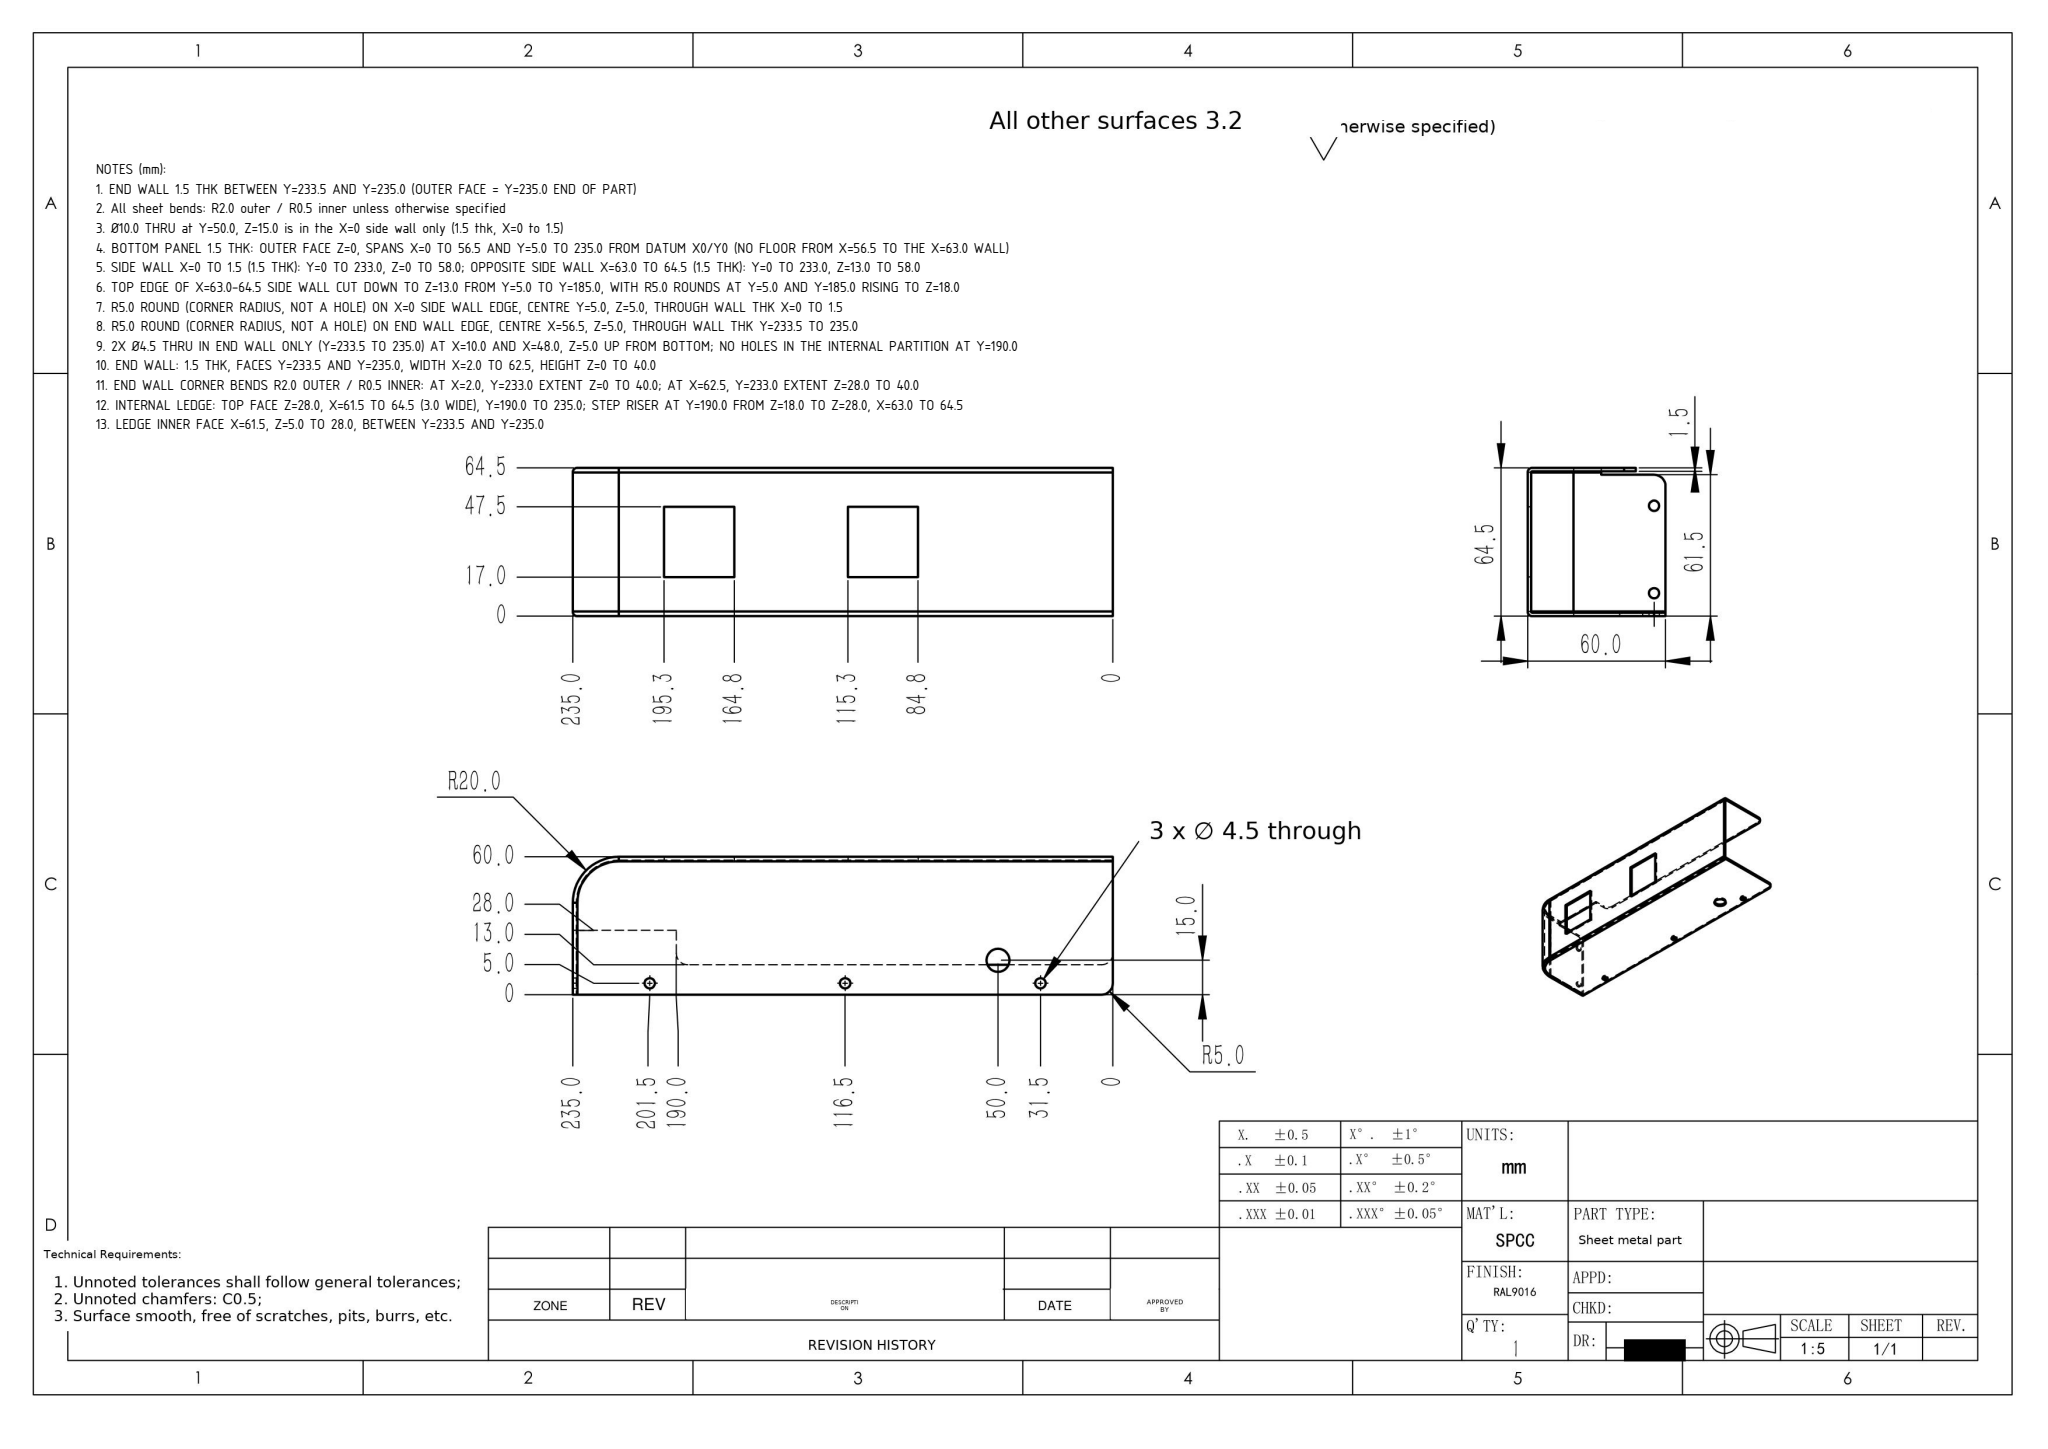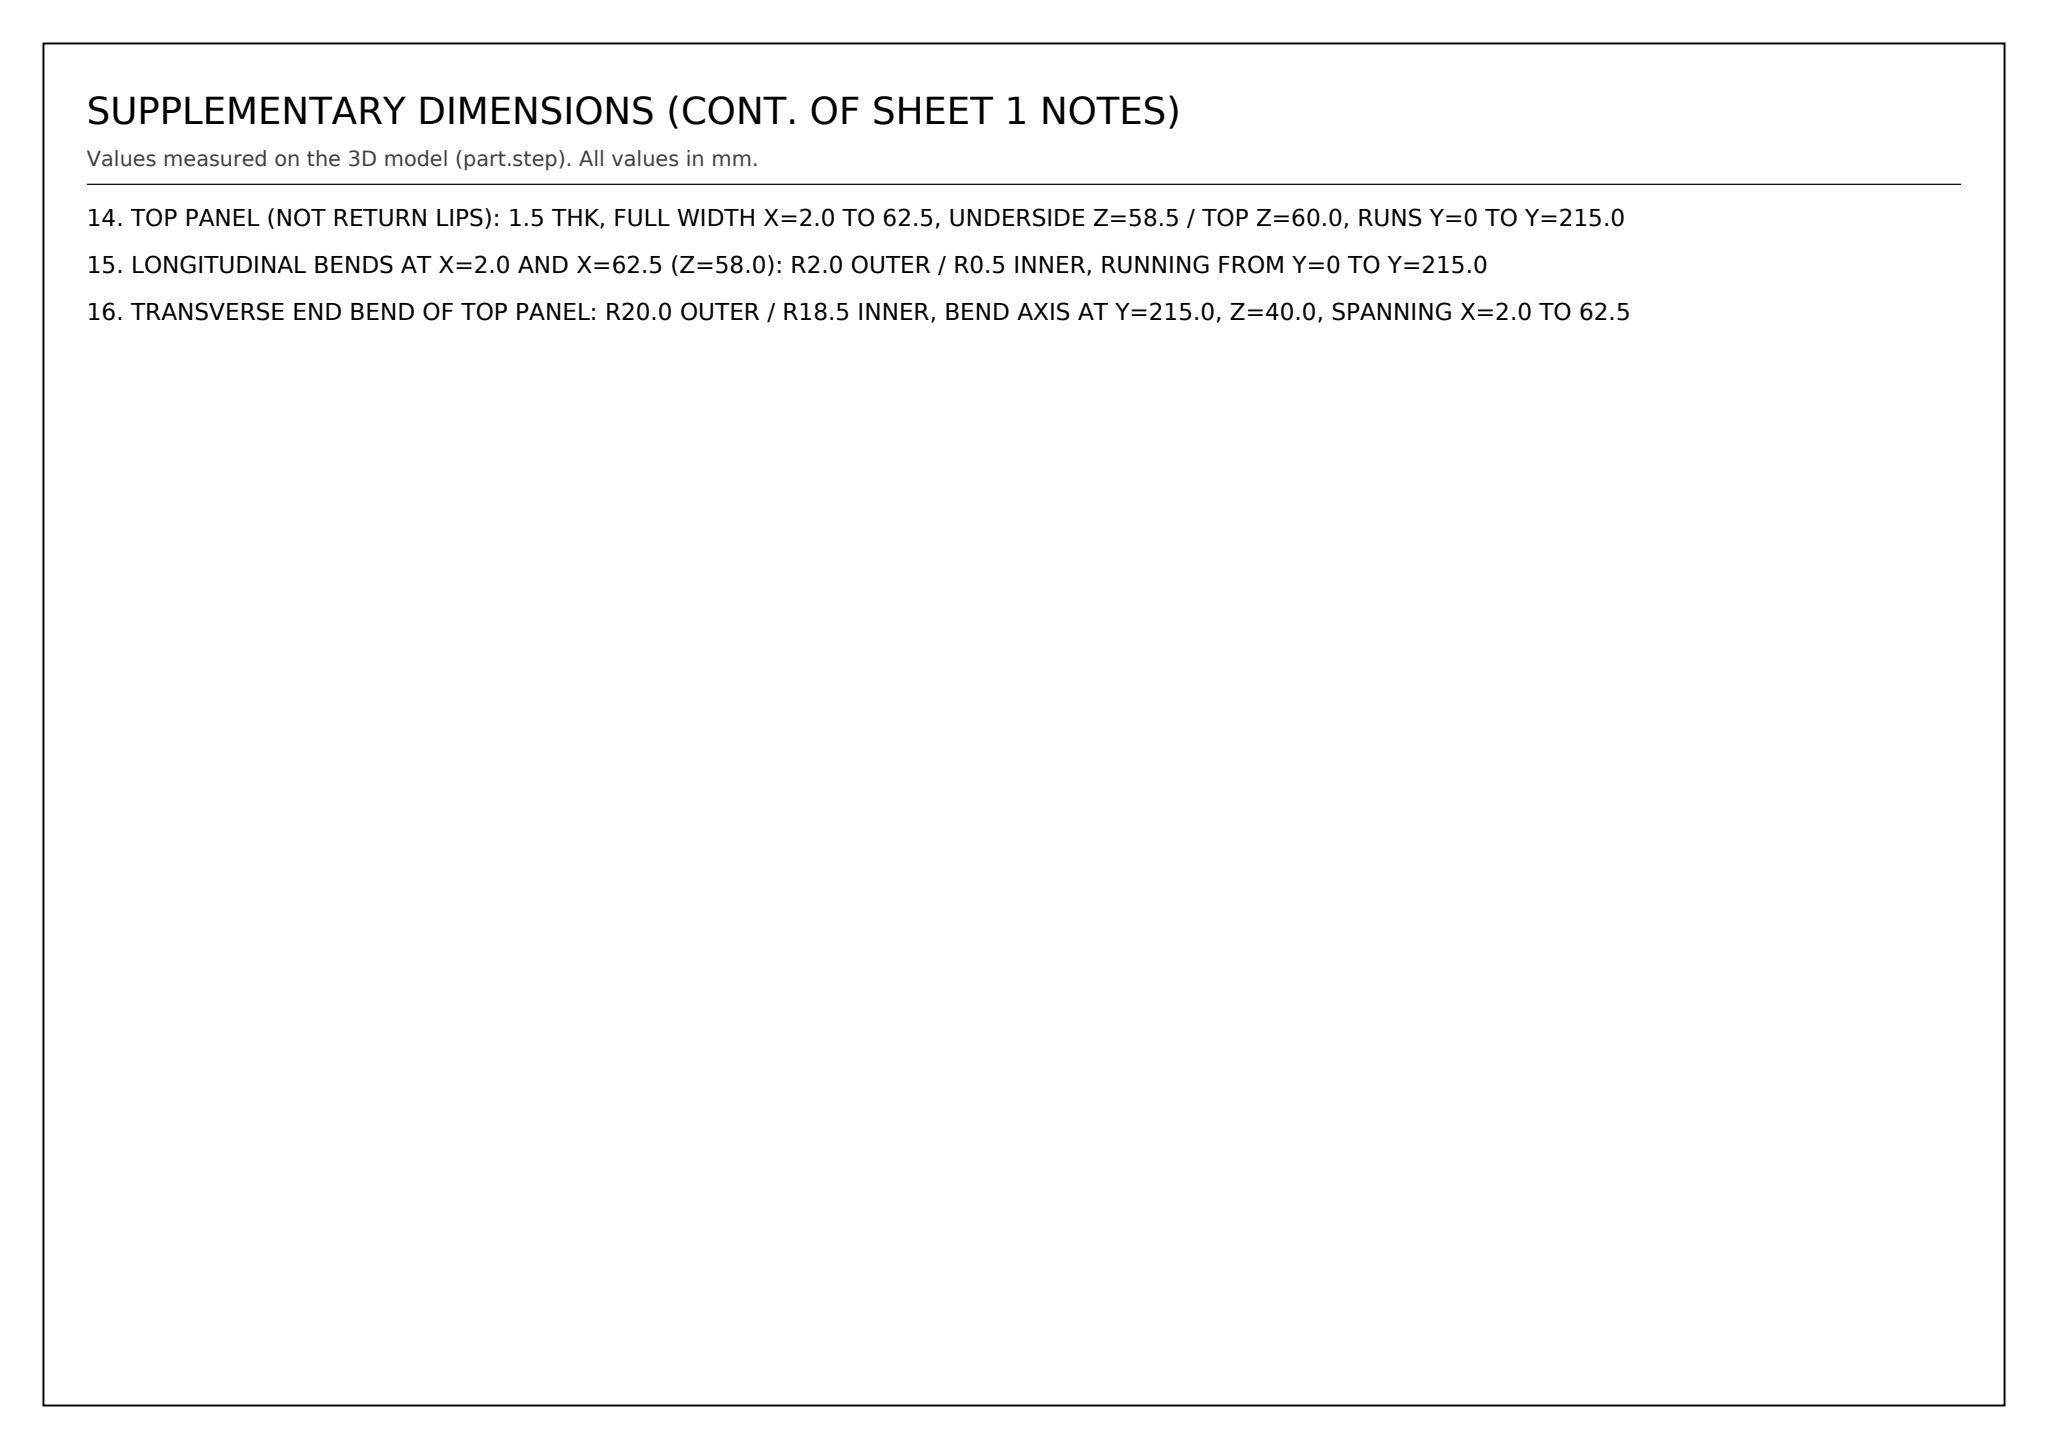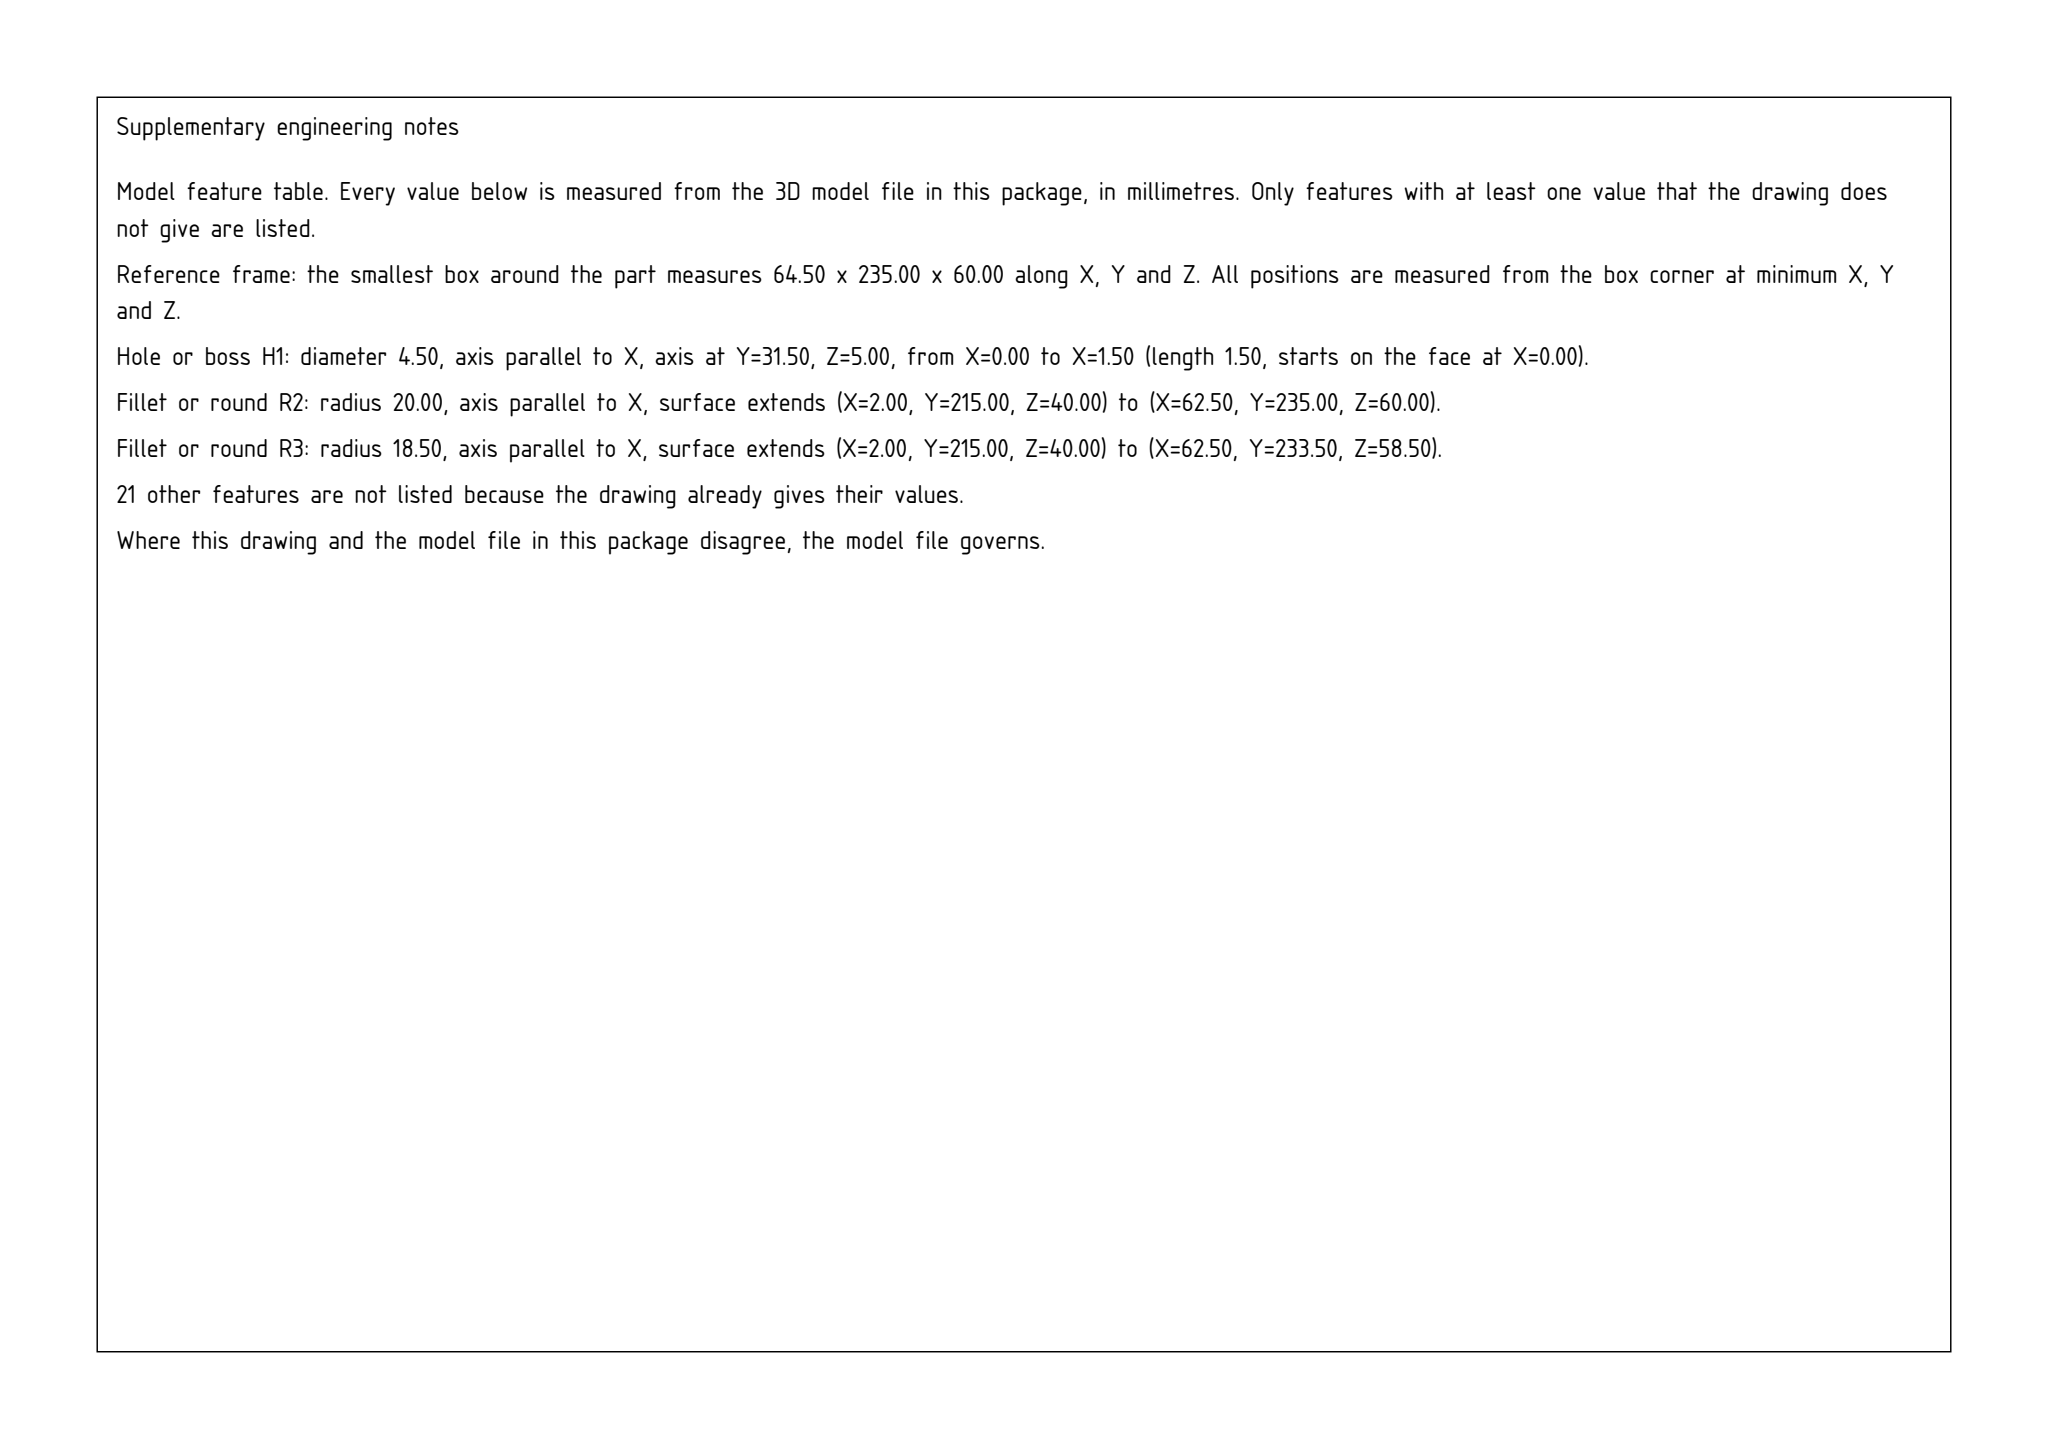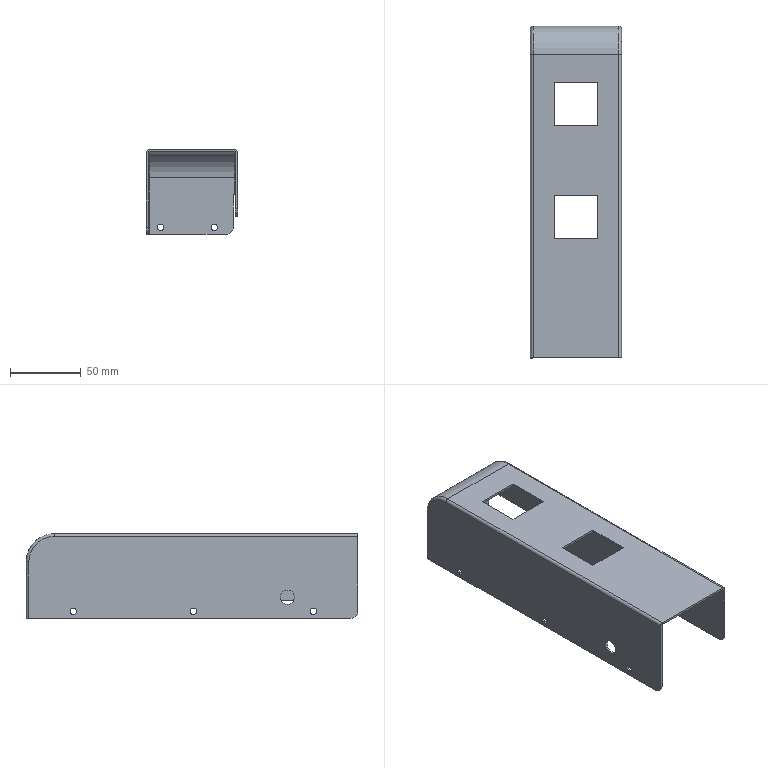Part | SolidWorks | mm | 1 solid | 52 faces | box 64.5 x 235 x 60 mm | volume 59200 mm3 | cylinder 26 | plane 22 | torus 4 | commonest cylinder face diameters 4.5 x10 10 x6 4 x4 1 x4 40 x1 37 x1
Drawing notes:
END WALL 1.5 THK BETWEEN Y=233.5 AND Y=235.0 (OUTER FACE = Y=235.0 END OF PART) | from the solid: axis_planes y 233.5 and y 235.0
All sheet bends: R2.0 outer / R0.5 inner unless otherwise specified | from the solid: fillet_radii [[2.0,2],[0.5,2]]
Ø10.0 THRU at Y=50.0, Z=15.0 is in the X=0 side wall only (1.5 thk, X=0 to 1.5) | from the solid: hole/bore dia 10.0, axis x, at (y=50.0, z=15.0), from x=0.0 to x=1.5, 360 deg
BOTTOM PANEL 1.5 THK: OUTER FACE Z=0, SPANS X=0 TO 56.5 AND Y=5.0 TO 235.0 FROM DATUM X0/Y0 (NO FLOOR FROM X=56.5 TO THE X=63.0 WALL) | from the solid: axis_plane z=0, extent x[0.0,56.5] y[5.0,235.0]
SIDE WALL X=0 TO 1.5 (1.5 THK): Y=0 TO 233.0, Z=0 TO 58.0; OPPOSITE SIDE WALL X=63.0 TO 64.5 (1.5 THK): Y=0 TO 233.0, Z=13.0 TO 58.0 | from the solid: axis_planes x=0.0 / x=1.5 (y[0,233], z[0,58]) and x=63.0 / x=64.5 (y[0,233], z[13,58])
TOP EDGE OF X=63.0-64.5 SIDE WALL CUT DOWN TO Z=13.0 FROM Y=5.0 TO Y=185.0, WITH R5.0 ROUNDS AT Y=5.0 AND Y=185.0 RISING TO Z=18.0 | from the solid: axis_plane z=13.0 x[63.0,64.5] y[5.0,185.0]; convex arcs Ø10.0 axis x at (y=5.0,z=18.0) and (y=185.0,z=18.0), x 63.0 to 64.5, 90°
R5.0 ROUND (CORNER RADIUS, NOT A HOLE) ON X=0 SIDE WALL EDGE, CENTRE Y=5.0, Z=5.0, THROUGH WALL THK X=0 TO 1.5 | from the solid: convex arc Ø10.0 axis x at (y=5.0, z=5.0), from x=0.0 to 1.5, 90°
R5.0 ROUND (CORNER RADIUS, NOT A HOLE) ON END WALL EDGE, CENTRE X=56.5, Z=5.0, THROUGH WALL THK Y=233.5 TO 235.0 | from the solid: convex arc Ø10.0 axis y at (x=56.5, z=5.0), from y=233.5 to 235.0, 90°
2X Ø4.5 THRU IN END WALL ONLY (Y=233.5 TO 235.0) AT X=10.0 AND X=48.0, Z=5.0 UP FROM BOTTOM; NO HOLES IN THE INTERNAL PARTITION AT Y=190.0 | from the solid: hole/bore Ø4.5 axis y at (x=10.0, z=5.0) and (x=48.0, z=5.0), y 233.5 to 235.0, 360°
END WALL: 1.5 THK, FACES Y=233.5 AND Y=235.0, WIDTH X=2.0 TO 62.5, HEIGHT Z=0 TO 40.0 | from the solid: axis_planes y=233.5 and y=235.0, extent x[2.0,62.5] z[0.0,40.0]
END WALL CORNER BENDS R2.0 OUTER / R0.5 INNER: AT X=2.0, Y=233.0 EXTENT Z=0 TO 40.0; AT X=62.5, Y=233.0 EXTENT Z=28.0 TO 40.0 | from the solid: concave Ø1.0 and convex Ø4.0 arcs axis z at (2.0,233.0) z 0 to 40.0 and at (62.5,233.0) z 28.0 to 40.0
INTERNAL LEDGE: TOP FACE Z=28.0, X=61.5 TO 64.5 (3.0 WIDE), Y=190.0 TO 235.0; STEP RISER AT Y=190.0 FROM Z=18.0 TO Z=28.0, X=63.0 TO 64.5 | from the solid: axis_plane z=28.0 x[61.5,64.5] y[190.0,235.0]; axis_plane y=190.0 x[63.0,64.5] z[18.0,28.0]
LEDGE INNER FACE X=61.5, Z=5.0 TO 28.0, BETWEEN Y=233.5 AND Y=235.0 | from the solid: axis_plane x=61.5, extent y[233.5,235.0] z[5.0,28.0]
TOP PANEL (NOT RETURN LIPS): 1.5 THK, FULL WIDTH X=2.0 TO 62.5, UNDERSIDE Z=58.5 / TOP Z=60.0, RUNS Y=0 TO Y=215.0 | from the solid: axis_planes z=58.5 and z=60.0, extent x[2.0,62.5] y[0.0,215.0]
LONGITUDINAL BENDS AT X=2.0 AND X=62.5 (Z=58.0): R2.0 OUTER / R0.5 INNER, RUNNING FROM Y=0 TO Y=215.0 | from the solid: concave Ø1.0 and convex Ø4.0 arcs axis y at (2.0,58.0) and (62.5,58.0), from y=0.0 to 215.0
TRANSVERSE END BEND OF TOP PANEL: R20.0 OUTER / R18.5 INNER, BEND AXIS AT Y=215.0, Z=40.0, SPANNING X=2.0 TO 62.5 | from the solid: convex arc Ø40.0 and concave arc Ø37.0, axis x at (y=215.0, z=40.0), x 2.0 to 62.5, 90°
build123d program:
from build123d import *

# Parameters (mm, degrees)
SKETCH1_W            = 64.5
SKETCH1_H            = 235
BOSS_EXTRUDE1_DEPTH  = 60
FILLET2_R            = 20
FILLET3_R            = 2
SHELL1_T             = -1.5
CUT_EXTRUDE1_REACH   = 246.673
SKETCH2_W            = 30.5
SKETCH2_H            = 30.5
CUT_EXTRUDE3_DEPTH   = 244.233
CUT_EXTRUDE5_DEPTH   = 3
M4_CLEARANCE_HOLE1_D = 4.5
CUT_EXTRUDE6_REACH   = 252.969
SKETCH8_R            = 5
M4_CLEARANCE_HOLE2_D = 4.5
FILLET4_R            = 5


with BuildPart() as part:
    # Sketch1 → Boss-Extrude1 (new body)
    with BuildSketch(Plane.XY):
        with Locations((0, 117.5)):
            Rectangle(SKETCH1_W, SKETCH1_H)
    extrude(amount=BOSS_EXTRUDE1_DEPTH)

    # Fillet2
    fillet2_edges = [part.edges().sort_by_distance(p)[0] for p in [
        (0, 235, 60),
    ]]
    fillet(fillet2_edges, radius=FILLET2_R)

    # Fillet3
    fillet3_edges = [part.edges().sort_by_distance(p)[0] for p in [
        (32.25, 107.5, 60),
        (-32.25, 107.5, 60),
        (-32.25, 235, 20),
        (-32.25, 229.142, 54.142),
        (32.25, 235, 20),
        (32.25, 229.142, 54.142),
    ]]
    fillet(fillet3_edges, radius=FILLET3_R)

    # Shell1
    shell1_openings = [part.faces().sort_by_distance(p)[0] for p in [
        (0, 117.487, 0),
    ]]
    offset(amount=SHELL1_T, openings=shell1_openings, kind=Kind.INTERSECTION)

    # Sketch2 → Cut-Extrude1 (cut, up to next)
    with BuildSketch(Plane.XY.offset(60), mode=Mode.PRIVATE) as cut_extrude1_sk1:
        with Locations((0, 180)):
            Rectangle(SKETCH2_W, SKETCH2_H)
    cut_extrude1_tool1 = extrude(cut_extrude1_sk1.sketch, amount=-CUT_EXTRUDE1_REACH, mode=Mode.PRIVATE) & part.part
    # Sketch2 → Cut-Extrude1 (cut, up to next)
    with BuildSketch(Plane.XY.offset(60), mode=Mode.PRIVATE) as cut_extrude1_sk2:
        with Locations((0, 100)):
            Rectangle(SKETCH2_W, SKETCH2_H)
    cut_extrude1_tool2 = extrude(cut_extrude1_sk2.sketch, amount=-CUT_EXTRUDE1_REACH, mode=Mode.PRIVATE) & part.part
    add(cut_extrude1_tool1.solids().sort_by_distance((0, 180, 60))[0], mode=Mode.SUBTRACT)
    add(cut_extrude1_tool2.solids().sort_by_distance((0, 100, 60))[0], mode=Mode.SUBTRACT)

    # Sketch4 → Cut-Extrude3 (cut, through all)
    with BuildSketch(Plane(origin=(0, 1.5, 0), x_dir=(1, 0, 0), z_dir=(0, 1, 0))):
        with BuildLine():
            Line((-30.25, -58.5), (30.25, -58.5))
            ThreePointArc((30.25, -58.5), (30.604, -58.354), (30.75, -58))
            Line((30.75, -58), (30.75, 0))
            Line((30.75, 0), (-30.75, 0))
            Line((-30.75, 0), (-30.75, -58))
            ThreePointArc((-30.75, -58), (-30.604, -58.354), (-30.25, -58.5))
        make_face()
    extrude(amount=-CUT_EXTRUDE3_DEPTH, mode=Mode.SUBTRACT)

    # Sketch5 → Cut-Extrude5 (cut)
    with BuildSketch(Plane(origin=(32.25, 0, 0), x_dir=(0, 0, -1), z_dir=(1, 0, 0))):
        Polygon((0, 0), (-13, 0), (-13, 190), (-28, 190), (-28, 235), (0, 235), align=None)
    extrude(amount=-CUT_EXTRUDE5_DEPTH, mode=Mode.SUBTRACT)

    # M4 Clearance Hole1 (through all)
    with Locations(Plane.ZY.offset(32.25)):
        with Locations((5, 31.5), (5, 201.5), (5, 116.5)):
            Hole(M4_CLEARANCE_HOLE1_D / 2)

    # Sketch8 → Cut-Extrude6 (cut, up to next)
    with BuildSketch(Plane.ZY.offset(32.25), mode=Mode.PRIVATE) as cut_extrude6_sk1:
        with Locations((15, 50)):
            Circle(SKETCH8_R)
    cut_extrude6_tool1 = extrude(cut_extrude6_sk1.sketch, amount=-CUT_EXTRUDE6_REACH, mode=Mode.PRIVATE) & part.part
    add(cut_extrude6_tool1.solids().sort_by_distance((-32.25, 50, 15))[0], mode=Mode.SUBTRACT)

    # M4 Clearance Hole2 (through all)
    with Locations(Plane(origin=(0, 235, 0), x_dir=(1, 0, 0), z_dir=(0, 1, 0))):
        with Locations((-22.25, -5), (15.75, -5)):
            Hole(M4_CLEARANCE_HOLE2_D / 2)

    # Fillet4
    fillet4_edges = [part.edges().sort_by_distance(p)[0] for p in [
        (29.25, 234.25, 0),
        (31.5, 0, 13),
        (31.5, 190, 13),
        (-31.5, 0, 0),
    ]]
    fillet(fillet4_edges, radius=FILLET4_R)


solid = part.part